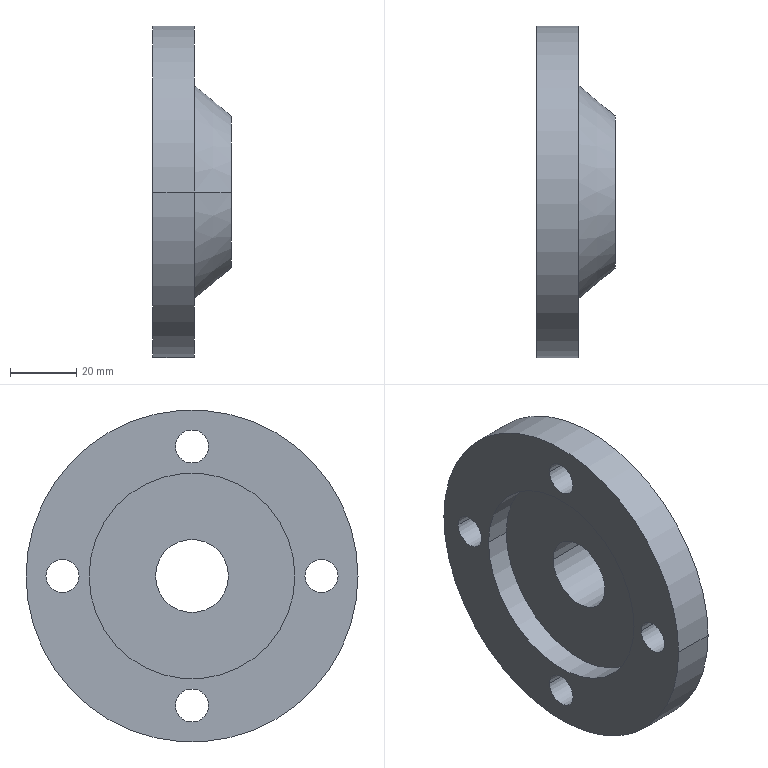Component | SolidWorks | RearEndCap-1 | 1 solid | 20 faces | box 23.63 x 100 x 100 mm | volume 92342 mm3 | cylinder 14 | plane 4 | cone 2 | commonest cylinder face diameters 10 x8 62 x2 100 x2 22 x2
build123d program:
from build123d import *

# Parameters (mm, degrees)
CUT_EXTRUDE1_DEPTH      = 211.672
CUT_EXTRUDE1_DEPTH_BACK = 211.672
SKETCH4_R               = 5
CUT_EXTRUDE2_START      = -5
SKETCH5_R               = 31
CUT_EXTRUDE2_DEPTH      = 10


with BuildPart() as part:
    # Sketch3 → Revolve1 (revolve)
    with BuildSketch(Plane(origin=(15, 0, 0), x_dir=(0, 0, -1), z_dir=(1, 0, 0)), mode=Mode.PRIVATE) as revolve1_sk:
        Polygon((0, 200), (-12.554, 200), (-12.554, 182.147), (-23.63, 172.896), (-23.63, 161), (0, 161), align=None)
    revolve(revolve1_sk.sketch.rotate(Axis((15, 150, 44.24), (0, 0, -1)), 90), axis=Axis((15, 150, 44.24), (0, 0, -1)))

    # Sketch4 → Cut-Extrude1 (cut, two sides: drawn at the far end of the back side and taken through both)
    with BuildSketch(Plane.XY.offset(12.554).offset(-CUT_EXTRUDE1_DEPTH_BACK)):
        with Locations((15, 189)):
            Circle(SKETCH4_R)
        with Locations((54, 150)):
            Circle(SKETCH4_R)
        with Locations((15, 111)):
            Circle(SKETCH4_R)
        with Locations((-24, 150)):
            Circle(SKETCH4_R)
    extrude(amount=CUT_EXTRUDE1_DEPTH + CUT_EXTRUDE1_DEPTH_BACK, mode=Mode.SUBTRACT)

    # Sketch5 → Cut-Extrude2 (cut)
    with BuildSketch(Plane.XY.offset(12.554).offset(CUT_EXTRUDE2_START)):
        with Locations((15, 150)):
            Circle(SKETCH5_R)
    extrude(amount=-CUT_EXTRUDE2_DEPTH, mode=Mode.SUBTRACT)


solid = part.part

# Placed as in the assembly
solid = solid.moved(Location((110, 0, 0), (0, 90, 0)))
STEP:
#1=COLOUR_RGB('',0.7922,0.8196,0.9333);
#2=FILL_AREA_STYLE_COLOUR('',#1);
#3=FILL_AREA_STYLE('',(#2));
#4=SURFACE_STYLE_FILL_AREA(#3);
#5=SURFACE_SIDE_STYLE('',(#4));
#6=SURFACE_STYLE_USAGE(.BOTH.,#5);
#7=PRESENTATION_STYLE_ASSIGNMENT((#6));
#8=CARTESIAN_POINT('',(4.331,7.126,-0.5906));
#9=VERTEX_POINT('',#8);
#10=CARTESIAN_POINT('',(4.331,4.685,-0.5906));
#11=VERTEX_POINT('',#10);
#12=CARTESIAN_POINT('',(4.331,5.906,-0.5906));
#13=DIRECTION('',(1.,0.,0.));
#14=DIRECTION('',(0.,-1.,-0.));
#15=AXIS2_PLACEMENT_3D('',#12,#13,#14);
#16=CIRCLE('',#15,1.22);
#17=EDGE_CURVE('',#9,#11,#16,.T.);
#18=ORIENTED_EDGE('',*,*,#17,.F.);
#19=CARTESIAN_POINT('',(4.628,7.126,-0.5906));
#20=VERTEX_POINT('',#19);
#21=CARTESIAN_POINT('',(4.234,7.126,-0.5906));
#22=DIRECTION('',(1.,0.,0.));
#23=VECTOR('',#22,39.37);
#24=LINE('',#21,#23);
#25=EDGE_CURVE('',#9,#20,#24,.T.);
#26=ORIENTED_EDGE('',*,*,#25,.T.);
#27=CARTESIAN_POINT('',(4.628,4.685,-0.5906));
#28=VERTEX_POINT('',#27);
#29=CARTESIAN_POINT('',(4.628,5.906,-0.5906));
#30=DIRECTION('',(1.,0.,0.));
#31=DIRECTION('',(0.,-1.,-0.));
#32=AXIS2_PLACEMENT_3D('',#29,#30,#31);
#33=CIRCLE('',#32,1.22);
#34=EDGE_CURVE('',#20,#28,#33,.T.);
#35=ORIENTED_EDGE('',*,*,#34,.T.);
#36=CARTESIAN_POINT('',(4.234,4.685,-0.5906));
#37=DIRECTION('',(1.,0.,0.));
#38=VECTOR('',#37,39.37);
#39=LINE('',#36,#38);
#40=EDGE_CURVE('',#11,#28,#39,.T.);
#41=ORIENTED_EDGE('',*,*,#40,.F.);
#42=EDGE_LOOP('',(#18,#26,#35,#41));
#43=FACE_OUTER_BOUND('',#42,.T.);
#44=CARTESIAN_POINT('',(4.234,5.906,-0.5906));
#45=DIRECTION('',(1.,0.,0.));
#46=DIRECTION('',(0.,-1.,-0.));
#47=AXIS2_PLACEMENT_3D('',#44,#45,#46);
#48=CYLINDRICAL_SURFACE('',#47,1.22);
#49=ADVANCED_FACE('',(#43),#48,.F.);
#50=CARTESIAN_POINT('',(4.331,6.102,-2.126));
#51=VERTEX_POINT('',#50);
#52=CARTESIAN_POINT('',(4.331,5.709,-2.126));
#53=VERTEX_POINT('',#52);
#54=CARTESIAN_POINT('',(4.331,5.906,-2.126));
#55=DIRECTION('',(1.,0.,0.));
#56=DIRECTION('',(0.,-1.,-0.));
#57=AXIS2_PLACEMENT_3D('',#54,#55,#56);
#58=CIRCLE('',#57,0.1969);
#59=EDGE_CURVE('',#51,#53,#58,.T.);
#60=ORIENTED_EDGE('',*,*,#59,.F.);
#61=CARTESIAN_POINT('',(4.825,6.102,-2.126));
#62=VERTEX_POINT('',#61);
#63=CARTESIAN_POINT('',(4.331,6.102,-2.126));
#64=DIRECTION('',(1.,0.,0.));
#65=VECTOR('',#64,39.37);
#66=LINE('',#63,#65);
#67=EDGE_CURVE('',#51,#62,#66,.T.);
#68=ORIENTED_EDGE('',*,*,#67,.T.);
#69=CARTESIAN_POINT('',(4.825,5.709,-2.126));
#70=VERTEX_POINT('',#69);
#71=CARTESIAN_POINT('',(4.825,5.906,-2.126));
#72=DIRECTION('',(-1.,-0.,-0.));
#73=DIRECTION('',(0.,1.,0.));
#74=AXIS2_PLACEMENT_3D('',#71,#72,#73);
#75=CIRCLE('',#74,0.1969);
#76=EDGE_CURVE('',#70,#62,#75,.T.);
#77=ORIENTED_EDGE('',*,*,#76,.F.);
#78=CARTESIAN_POINT('',(4.331,5.709,-2.126));
#79=DIRECTION('',(1.,0.,0.));
#80=VECTOR('',#79,39.37);
#81=LINE('',#78,#80);
#82=EDGE_CURVE('',#53,#70,#81,.T.);
#83=ORIENTED_EDGE('',*,*,#82,.F.);
#84=EDGE_LOOP('',(#60,#68,#77,#83));
#85=FACE_OUTER_BOUND('',#84,.T.);
#86=CARTESIAN_POINT('',(4.331,5.906,-2.126));
#87=DIRECTION('',(1.,0.,0.));
#88=DIRECTION('',(0.,-1.,-0.));
#89=AXIS2_PLACEMENT_3D('',#86,#87,#88);
#90=CYLINDRICAL_SURFACE('',#89,0.1969);
#91=ADVANCED_FACE('',(#85),#90,.F.);
#92=CARTESIAN_POINT('',(4.331,4.567,-0.5906));
#93=VERTEX_POINT('',#92);
#94=CARTESIAN_POINT('',(4.331,4.173,-0.5906));
#95=VERTEX_POINT('',#94);
#96=CARTESIAN_POINT('',(4.331,4.37,-0.5906));
#97=DIRECTION('',(1.,0.,0.));
#98=DIRECTION('',(0.,-1.,-0.));
#99=AXIS2_PLACEMENT_3D('',#96,#97,#98);
#100=CIRCLE('',#99,0.1969);
#101=EDGE_CURVE('',#93,#95,#100,.T.);
#102=ORIENTED_EDGE('',*,*,#101,.F.);
#103=CARTESIAN_POINT('',(4.825,4.567,-0.5906));
#104=VERTEX_POINT('',#103);
#105=CARTESIAN_POINT('',(4.331,4.567,-0.5906));
#106=DIRECTION('',(1.,0.,0.));
#107=VECTOR('',#106,39.37);
#108=LINE('',#105,#107);
#109=EDGE_CURVE('',#93,#104,#108,.T.);
#110=ORIENTED_EDGE('',*,*,#109,.T.);
#111=CARTESIAN_POINT('',(4.825,4.173,-0.5906));
#112=VERTEX_POINT('',#111);
#113=CARTESIAN_POINT('',(4.825,4.37,-0.5906));
#114=DIRECTION('',(-1.,-0.,-0.));
#115=DIRECTION('',(0.,1.,0.));
#116=AXIS2_PLACEMENT_3D('',#113,#114,#115);
#117=CIRCLE('',#116,0.1969);
#118=EDGE_CURVE('',#112,#104,#117,.T.);
#119=ORIENTED_EDGE('',*,*,#118,.F.);
#120=CARTESIAN_POINT('',(4.331,4.173,-0.5906));
#121=DIRECTION('',(1.,0.,0.));
#122=VECTOR('',#121,39.37);
#123=LINE('',#120,#122);
#124=EDGE_CURVE('',#95,#112,#123,.T.);
#125=ORIENTED_EDGE('',*,*,#124,.F.);
#126=EDGE_LOOP('',(#102,#110,#119,#125));
#127=FACE_OUTER_BOUND('',#126,.T.);
#128=CARTESIAN_POINT('',(4.331,4.37,-0.5906));
#129=DIRECTION('',(1.,0.,0.));
#130=DIRECTION('',(0.,-1.,-0.));
#131=AXIS2_PLACEMENT_3D('',#128,#129,#130);
#132=CYLINDRICAL_SURFACE('',#131,0.1969);
#133=ADVANCED_FACE('',(#127),#132,.F.);
#134=CARTESIAN_POINT('',(4.331,6.102,0.9449));
#135=VERTEX_POINT('',#134);
#136=CARTESIAN_POINT('',(4.331,5.709,0.9449));
#137=VERTEX_POINT('',#136);
#138=CARTESIAN_POINT('',(4.331,5.906,0.9449));
#139=DIRECTION('',(1.,0.,0.));
#140=DIRECTION('',(0.,-1.,-0.));
#141=AXIS2_PLACEMENT_3D('',#138,#139,#140);
#142=CIRCLE('',#141,0.1969);
#143=EDGE_CURVE('',#135,#137,#142,.T.);
#144=ORIENTED_EDGE('',*,*,#143,.F.);
#145=CARTESIAN_POINT('',(4.825,6.102,0.9449));
#146=VERTEX_POINT('',#145);
#147=CARTESIAN_POINT('',(4.331,6.102,0.9449));
#148=DIRECTION('',(1.,0.,0.));
#149=VECTOR('',#148,39.37);
#150=LINE('',#147,#149);
#151=EDGE_CURVE('',#135,#146,#150,.T.);
#152=ORIENTED_EDGE('',*,*,#151,.T.);
#153=CARTESIAN_POINT('',(4.825,5.709,0.9449));
#154=VERTEX_POINT('',#153);
#155=CARTESIAN_POINT('',(4.825,5.906,0.9449));
#156=DIRECTION('',(-1.,-0.,-0.));
#157=DIRECTION('',(0.,1.,0.));
#158=AXIS2_PLACEMENT_3D('',#155,#156,#157);
#159=CIRCLE('',#158,0.1969);
#160=EDGE_CURVE('',#154,#146,#159,.T.);
#161=ORIENTED_EDGE('',*,*,#160,.F.);
#162=CARTESIAN_POINT('',(4.331,5.709,0.9449));
#163=DIRECTION('',(1.,0.,0.));
#164=VECTOR('',#163,39.37);
#165=LINE('',#162,#164);
#166=EDGE_CURVE('',#137,#154,#165,.T.);
#167=ORIENTED_EDGE('',*,*,#166,.F.);
#168=EDGE_LOOP('',(#144,#152,#161,#167));
#169=FACE_OUTER_BOUND('',#168,.T.);
#170=CARTESIAN_POINT('',(4.331,5.906,0.9449));
#171=DIRECTION('',(1.,0.,0.));
#172=DIRECTION('',(0.,-1.,-0.));
#173=AXIS2_PLACEMENT_3D('',#170,#171,#172);
#174=CYLINDRICAL_SURFACE('',#173,0.1969);
#175=ADVANCED_FACE('',(#169),#174,.F.);
#176=CARTESIAN_POINT('',(4.331,7.638,-0.5906));
#177=VERTEX_POINT('',#176);
#178=CARTESIAN_POINT('',(4.331,7.244,-0.5906));
#179=VERTEX_POINT('',#178);
#180=CARTESIAN_POINT('',(4.331,7.441,-0.5906));
#181=DIRECTION('',(1.,0.,0.));
#182=DIRECTION('',(0.,-1.,-0.));
#183=AXIS2_PLACEMENT_3D('',#180,#181,#182);
#184=CIRCLE('',#183,0.1969);
#185=EDGE_CURVE('',#177,#179,#184,.T.);
#186=ORIENTED_EDGE('',*,*,#185,.F.);
#187=CARTESIAN_POINT('',(4.825,7.638,-0.5906));
#188=VERTEX_POINT('',#187);
#189=CARTESIAN_POINT('',(4.331,7.638,-0.5906));
#190=DIRECTION('',(1.,0.,0.));
#191=VECTOR('',#190,39.37);
#192=LINE('',#189,#191);
#193=EDGE_CURVE('',#177,#188,#192,.T.);
#194=ORIENTED_EDGE('',*,*,#193,.T.);
#195=CARTESIAN_POINT('',(4.825,7.244,-0.5906));
#196=VERTEX_POINT('',#195);
#197=CARTESIAN_POINT('',(4.825,7.441,-0.5906));
#198=DIRECTION('',(-1.,-0.,-0.));
#199=DIRECTION('',(0.,1.,0.));
#200=AXIS2_PLACEMENT_3D('',#197,#198,#199);
#201=CIRCLE('',#200,0.1969);
#202=EDGE_CURVE('',#196,#188,#201,.T.);
#203=ORIENTED_EDGE('',*,*,#202,.F.);
#204=CARTESIAN_POINT('',(4.331,7.244,-0.5906));
#205=DIRECTION('',(1.,0.,0.));
#206=VECTOR('',#205,39.37);
#207=LINE('',#204,#206);
#208=EDGE_CURVE('',#179,#196,#207,.T.);
#209=ORIENTED_EDGE('',*,*,#208,.F.);
#210=EDGE_LOOP('',(#186,#194,#203,#209));
#211=FACE_OUTER_BOUND('',#210,.T.);
#212=CARTESIAN_POINT('',(4.331,7.441,-0.5906));
#213=DIRECTION('',(1.,0.,0.));
#214=DIRECTION('',(0.,-1.,-0.));
#215=AXIS2_PLACEMENT_3D('',#212,#213,#214);
#216=CYLINDRICAL_SURFACE('',#215,0.1969);
#217=ADVANCED_FACE('',(#211),#216,.F.);
#218=CARTESIAN_POINT('',(4.331,3.937,-0.5906));
#219=VERTEX_POINT('',#218);
#220=CARTESIAN_POINT('',(4.331,7.874,-0.5906));
#221=VERTEX_POINT('',#220);
#222=CARTESIAN_POINT('',(4.331,5.906,-0.5906));
#223=DIRECTION('',(1.,0.,0.));
#224=DIRECTION('',(0.,-1.,-0.));
#225=AXIS2_PLACEMENT_3D('',#222,#223,#224);
#226=CIRCLE('',#225,1.969);
#227=EDGE_CURVE('',#219,#221,#226,.T.);
#228=ORIENTED_EDGE('',*,*,#227,.T.);
#229=CARTESIAN_POINT('',(4.825,7.874,-0.5906));
#230=VERTEX_POINT('',#229);
#231=CARTESIAN_POINT('',(6.072,7.874,-0.5906));
#232=DIRECTION('',(1.,0.,0.));
#233=VECTOR('',#232,39.37);
#234=LINE('',#231,#233);
#235=EDGE_CURVE('',#221,#230,#234,.T.);
#236=ORIENTED_EDGE('',*,*,#235,.T.);
#237=CARTESIAN_POINT('',(4.825,3.937,-0.5906));
#238=VERTEX_POINT('',#237);
#239=CARTESIAN_POINT('',(4.825,5.906,-0.5906));
#240=DIRECTION('',(1.,0.,0.));
#241=DIRECTION('',(0.,-1.,-0.));
#242=AXIS2_PLACEMENT_3D('',#239,#240,#241);
#243=CIRCLE('',#242,1.969);
#244=EDGE_CURVE('',#238,#230,#243,.T.);
#245=ORIENTED_EDGE('',*,*,#244,.F.);
#246=CARTESIAN_POINT('',(6.072,3.937,-0.5906));
#247=DIRECTION('',(1.,0.,0.));
#248=VECTOR('',#247,39.37);
#249=LINE('',#246,#248);
#250=EDGE_CURVE('',#219,#238,#249,.T.);
#251=ORIENTED_EDGE('',*,*,#250,.F.);
#252=EDGE_LOOP('',(#228,#236,#245,#251));
#253=FACE_OUTER_BOUND('',#252,.T.);
#254=CARTESIAN_POINT('',(6.072,5.906,-0.5906));
#255=DIRECTION('',(1.,0.,0.));
#256=DIRECTION('',(0.,-1.,-0.));
#257=AXIS2_PLACEMENT_3D('',#254,#255,#256);
#258=CYLINDRICAL_SURFACE('',#257,1.969);
#259=ADVANCED_FACE('',(#253),#258,.T.);
#260=CARTESIAN_POINT('',(5.261,5.004,-0.5906));
#261=VERTEX_POINT('',#260);
#262=CARTESIAN_POINT('',(5.261,6.807,-0.5906));
#263=VERTEX_POINT('',#262);
#264=CARTESIAN_POINT('',(5.261,5.906,-0.5906));
#265=DIRECTION('',(1.,0.,0.));
#266=DIRECTION('',(0.,-1.,-0.));
#267=AXIS2_PLACEMENT_3D('',#264,#265,#266);
#268=CIRCLE('',#267,0.9014);
#269=EDGE_CURVE('',#261,#263,#268,.T.);
#270=ORIENTED_EDGE('',*,*,#269,.F.);
#271=CARTESIAN_POINT('',(4.825,4.64,-0.5906));
#272=VERTEX_POINT('',#271);
#273=CARTESIAN_POINT('',(4.825,4.64,-0.5906));
#274=DIRECTION('',(-0.7675,-0.641,-0.));
#275=VECTOR('',#274,39.37);
#276=LINE('',#273,#275);
#277=EDGE_CURVE('',#261,#272,#276,.T.);
#278=ORIENTED_EDGE('',*,*,#277,.T.);
#279=CARTESIAN_POINT('',(4.825,7.171,-0.5906));
#280=VERTEX_POINT('',#279);
#281=CARTESIAN_POINT('',(4.825,5.906,-0.5906));
#282=DIRECTION('',(1.,0.,0.));
#283=DIRECTION('',(0.,-1.,-0.));
#284=AXIS2_PLACEMENT_3D('',#281,#282,#283);
#285=CIRCLE('',#284,1.266);
#286=EDGE_CURVE('',#272,#280,#285,.T.);
#287=ORIENTED_EDGE('',*,*,#286,.T.);
#288=CARTESIAN_POINT('',(4.825,7.171,-0.5906));
#289=DIRECTION('',(-0.7675,0.641,0.));
#290=VECTOR('',#289,39.37);
#291=LINE('',#288,#290);
#292=EDGE_CURVE('',#263,#280,#291,.T.);
#293=ORIENTED_EDGE('',*,*,#292,.F.);
#294=EDGE_LOOP('',(#270,#278,#287,#293));
#295=FACE_OUTER_BOUND('',#294,.T.);
#296=CARTESIAN_POINT('',(4.825,5.906,-0.5906));
#297=DIRECTION('',(-1.,-0.,-0.));
#298=DIRECTION('',(0.,1.,0.));
#299=AXIS2_PLACEMENT_3D('',#296,#297,#298);
#300=CONICAL_SURFACE('',#299,1.266,0.6959);
#301=ADVANCED_FACE('',(#295),#300,.T.);
#302=CARTESIAN_POINT('',(4.628,5.472,-0.5906));
#303=VERTEX_POINT('',#302);
#304=CARTESIAN_POINT('',(4.628,6.339,-0.5906));
#305=VERTEX_POINT('',#304);
#306=CARTESIAN_POINT('',(4.628,5.906,-0.5906));
#307=DIRECTION('',(-1.,-0.,-0.));
#308=DIRECTION('',(0.,-1.,-0.));
#309=AXIS2_PLACEMENT_3D('',#306,#307,#308);
#310=CIRCLE('',#309,0.4331);
#311=EDGE_CURVE('',#303,#305,#310,.T.);
#312=ORIENTED_EDGE('',*,*,#311,.T.);
#313=CARTESIAN_POINT('',(5.261,6.339,-0.5906));
#314=VERTEX_POINT('',#313);
#315=CARTESIAN_POINT('',(6.072,6.339,-0.5906));
#316=DIRECTION('',(1.,0.,0.));
#317=VECTOR('',#316,39.37);
#318=LINE('',#315,#317);
#319=EDGE_CURVE('',#305,#314,#318,.T.);
#320=ORIENTED_EDGE('',*,*,#319,.T.);
#321=CARTESIAN_POINT('',(5.261,5.472,-0.5906));
#322=VERTEX_POINT('',#321);
#323=CARTESIAN_POINT('',(5.261,5.906,-0.5906));
#324=DIRECTION('',(1.,0.,0.));
#325=DIRECTION('',(0.,-1.,-0.));
#326=AXIS2_PLACEMENT_3D('',#323,#324,#325);
#327=CIRCLE('',#326,0.4331);
#328=EDGE_CURVE('',#314,#322,#327,.T.);
#329=ORIENTED_EDGE('',*,*,#328,.T.);
#330=CARTESIAN_POINT('',(6.072,5.472,-0.5906));
#331=DIRECTION('',(1.,0.,0.));
#332=VECTOR('',#331,39.37);
#333=LINE('',#330,#332);
#334=EDGE_CURVE('',#303,#322,#333,.T.);
#335=ORIENTED_EDGE('',*,*,#334,.F.);
#336=EDGE_LOOP('',(#312,#320,#329,#335));
#337=FACE_OUTER_BOUND('',#336,.T.);
#338=CARTESIAN_POINT('',(6.072,5.906,-0.5906));
#339=DIRECTION('',(1.,0.,0.));
#340=DIRECTION('',(0.,-1.,-0.));
#341=AXIS2_PLACEMENT_3D('',#338,#339,#340);
#342=CYLINDRICAL_SURFACE('',#341,0.4331);
#343=ADVANCED_FACE('',(#337),#342,.F.);
#344=CARTESIAN_POINT('',(4.331,5.906,-0.5906));
#345=DIRECTION('',(1.,0.,0.));
#346=DIRECTION('',(0.,-1.,-0.));
#347=AXIS2_PLACEMENT_3D('',#344,#345,#346);
#348=CIRCLE('',#347,1.22);
#349=EDGE_CURVE('',#11,#9,#348,.T.);
#350=ORIENTED_EDGE('',*,*,#349,.T.);
#351=ORIENTED_EDGE('',*,*,#17,.T.);
#352=EDGE_LOOP('',(#350,#351));
#353=FACE_BOUND('',#352,.T.);
#354=CARTESIAN_POINT('',(4.331,5.906,-2.126));
#355=DIRECTION('',(1.,0.,0.));
#356=DIRECTION('',(0.,-1.,-0.));
#357=AXIS2_PLACEMENT_3D('',#354,#355,#356);
#358=CIRCLE('',#357,0.1969);
#359=EDGE_CURVE('',#53,#51,#358,.T.);
#360=ORIENTED_EDGE('',*,*,#359,.T.);
#361=ORIENTED_EDGE('',*,*,#59,.T.);
#362=EDGE_LOOP('',(#360,#361));
#363=FACE_BOUND('',#362,.T.);
#364=CARTESIAN_POINT('',(4.331,4.37,-0.5906));
#365=DIRECTION('',(1.,0.,0.));
#366=DIRECTION('',(0.,-1.,-0.));
#367=AXIS2_PLACEMENT_3D('',#364,#365,#366);
#368=CIRCLE('',#367,0.1969);
#369=EDGE_CURVE('',#95,#93,#368,.T.);
#370=ORIENTED_EDGE('',*,*,#369,.T.);
#371=ORIENTED_EDGE('',*,*,#101,.T.);
#372=EDGE_LOOP('',(#370,#371));
#373=FACE_BOUND('',#372,.T.);
#374=CARTESIAN_POINT('',(4.331,5.906,0.9449));
#375=DIRECTION('',(1.,0.,0.));
#376=DIRECTION('',(0.,-1.,-0.));
#377=AXIS2_PLACEMENT_3D('',#374,#375,#376);
#378=CIRCLE('',#377,0.1969);
#379=EDGE_CURVE('',#137,#135,#378,.T.);
#380=ORIENTED_EDGE('',*,*,#379,.T.);
#381=ORIENTED_EDGE('',*,*,#143,.T.);
#382=EDGE_LOOP('',(#380,#381));
#383=FACE_BOUND('',#382,.T.);
#384=CARTESIAN_POINT('',(4.331,7.441,-0.5906));
#385=DIRECTION('',(1.,0.,0.));
#386=DIRECTION('',(0.,-1.,-0.));
#387=AXIS2_PLACEMENT_3D('',#384,#385,#386);
#388=CIRCLE('',#387,0.1969);
#389=EDGE_CURVE('',#179,#177,#388,.T.);
#390=ORIENTED_EDGE('',*,*,#389,.T.);
#391=ORIENTED_EDGE('',*,*,#185,.T.);
#392=EDGE_LOOP('',(#390,#391));
#393=FACE_BOUND('',#392,.T.);
#394=ORIENTED_EDGE('',*,*,#227,.F.);
#395=CARTESIAN_POINT('',(4.331,5.906,-0.5906));
#396=DIRECTION('',(1.,0.,0.));
#397=DIRECTION('',(0.,-1.,-0.));
#398=AXIS2_PLACEMENT_3D('',#395,#396,#397);
#399=CIRCLE('',#398,1.969);
#400=EDGE_CURVE('',#221,#219,#399,.T.);
#401=ORIENTED_EDGE('',*,*,#400,.F.);
#402=EDGE_LOOP('',(#394,#401));
#403=FACE_OUTER_BOUND('',#402,.T.);
#404=CARTESIAN_POINT('',(4.331,5.906,-2.559));
#405=DIRECTION('',(1.,0.,0.));
#406=DIRECTION('',(0.,-1.,-0.));
#407=AXIS2_PLACEMENT_3D('',#404,#405,#406);
#408=PLANE('',#407);
#409=ADVANCED_FACE('',(#353,#363,#373,#383,#393,#403),#408,.F.);
#410=ORIENTED_EDGE('',*,*,#319,.F.);
#411=CARTESIAN_POINT('',(4.628,5.906,-0.5906));
#412=DIRECTION('',(-1.,-0.,-0.));
#413=DIRECTION('',(0.,-1.,-0.));
#414=AXIS2_PLACEMENT_3D('',#411,#412,#413);
#415=CIRCLE('',#414,0.4331);
#416=EDGE_CURVE('',#305,#303,#415,.T.);
#417=ORIENTED_EDGE('',*,*,#416,.T.);
#418=ORIENTED_EDGE('',*,*,#334,.T.);
#419=CARTESIAN_POINT('',(5.261,5.906,-0.5906));
#420=DIRECTION('',(1.,0.,0.));
#421=DIRECTION('',(0.,-1.,-0.));
#422=AXIS2_PLACEMENT_3D('',#419,#420,#421);
#423=CIRCLE('',#422,0.4331);
#424=EDGE_CURVE('',#322,#314,#423,.T.);
#425=ORIENTED_EDGE('',*,*,#424,.T.);
#426=EDGE_LOOP('',(#410,#417,#418,#425));
#427=FACE_OUTER_BOUND('',#426,.T.);
#428=CARTESIAN_POINT('',(6.072,5.906,-0.5906));
#429=DIRECTION('',(1.,0.,0.));
#430=DIRECTION('',(0.,-1.,-0.));
#431=AXIS2_PLACEMENT_3D('',#428,#429,#430);
#432=CYLINDRICAL_SURFACE('',#431,0.4331);
#433=ADVANCED_FACE('',(#427),#432,.F.);
#434=ORIENTED_EDGE('',*,*,#424,.F.);
#435=ORIENTED_EDGE('',*,*,#328,.F.);
#436=EDGE_LOOP('',(#434,#435));
#437=FACE_BOUND('',#436,.T.);
#438=CARTESIAN_POINT('',(5.261,5.906,-0.5906));
#439=DIRECTION('',(1.,0.,0.));
#440=DIRECTION('',(0.,-1.,-0.));
#441=AXIS2_PLACEMENT_3D('',#438,#439,#440);
#442=CIRCLE('',#441,0.9014);
#443=EDGE_CURVE('',#263,#261,#442,.T.);
#444=ORIENTED_EDGE('',*,*,#443,.T.);
#445=ORIENTED_EDGE('',*,*,#269,.T.);
#446=EDGE_LOOP('',(#444,#445));
#447=FACE_OUTER_BOUND('',#446,.T.);
#448=CARTESIAN_POINT('',(5.261,5.906,-1.492));
#449=DIRECTION('',(-1.,-0.,-0.));
#450=DIRECTION('',(-0.,1.,0.));
#451=AXIS2_PLACEMENT_3D('',#448,#449,#450);
#452=PLANE('',#451);
#453=ADVANCED_FACE('',(#437,#447),#452,.F.);
#454=ORIENTED_EDGE('',*,*,#277,.F.);
#455=ORIENTED_EDGE('',*,*,#443,.F.);
#456=ORIENTED_EDGE('',*,*,#292,.T.);
#457=CARTESIAN_POINT('',(4.825,5.906,-0.5906));
#458=DIRECTION('',(1.,0.,0.));
#459=DIRECTION('',(0.,-1.,-0.));
#460=AXIS2_PLACEMENT_3D('',#457,#458,#459);
#461=CIRCLE('',#460,1.266);
#462=EDGE_CURVE('',#280,#272,#461,.T.);
#463=ORIENTED_EDGE('',*,*,#462,.T.);
#464=EDGE_LOOP('',(#454,#455,#456,#463));
#465=FACE_OUTER_BOUND('',#464,.T.);
#466=CARTESIAN_POINT('',(4.825,5.906,-0.5906));
#467=DIRECTION('',(-1.,-0.,-0.));
#468=DIRECTION('',(0.,1.,0.));
#469=AXIS2_PLACEMENT_3D('',#466,#467,#468);
#470=CONICAL_SURFACE('',#469,1.266,0.6959);
#471=ADVANCED_FACE('',(#465),#470,.T.);
#472=ORIENTED_EDGE('',*,*,#76,.T.);
#473=CARTESIAN_POINT('',(4.825,5.906,-2.126));
#474=DIRECTION('',(-1.,-0.,-0.));
#475=DIRECTION('',(0.,1.,0.));
#476=AXIS2_PLACEMENT_3D('',#473,#474,#475);
#477=CIRCLE('',#476,0.1969);
#478=EDGE_CURVE('',#62,#70,#477,.T.);
#479=ORIENTED_EDGE('',*,*,#478,.T.);
#480=EDGE_LOOP('',(#472,#479));
#481=FACE_BOUND('',#480,.T.);
#482=ORIENTED_EDGE('',*,*,#118,.T.);
#483=CARTESIAN_POINT('',(4.825,4.37,-0.5906));
#484=DIRECTION('',(-1.,-0.,-0.));
#485=DIRECTION('',(0.,1.,0.));
#486=AXIS2_PLACEMENT_3D('',#483,#484,#485);
#487=CIRCLE('',#486,0.1969);
#488=EDGE_CURVE('',#104,#112,#487,.T.);
#489=ORIENTED_EDGE('',*,*,#488,.T.);
#490=EDGE_LOOP('',(#482,#489));
#491=FACE_BOUND('',#490,.T.);
#492=ORIENTED_EDGE('',*,*,#160,.T.);
#493=CARTESIAN_POINT('',(4.825,5.906,0.9449));
#494=DIRECTION('',(-1.,-0.,-0.));
#495=DIRECTION('',(0.,1.,0.));
#496=AXIS2_PLACEMENT_3D('',#493,#494,#495);
#497=CIRCLE('',#496,0.1969);
#498=EDGE_CURVE('',#146,#154,#497,.T.);
#499=ORIENTED_EDGE('',*,*,#498,.T.);
#500=EDGE_LOOP('',(#492,#499));
#501=FACE_BOUND('',#500,.T.);
#502=ORIENTED_EDGE('',*,*,#202,.T.);
#503=CARTESIAN_POINT('',(4.825,7.441,-0.5906));
#504=DIRECTION('',(-1.,-0.,-0.));
#505=DIRECTION('',(0.,1.,0.));
#506=AXIS2_PLACEMENT_3D('',#503,#504,#505);
#507=CIRCLE('',#506,0.1969);
#508=EDGE_CURVE('',#188,#196,#507,.T.);
#509=ORIENTED_EDGE('',*,*,#508,.T.);
#510=EDGE_LOOP('',(#502,#509));
#511=FACE_BOUND('',#510,.T.);
#512=ORIENTED_EDGE('',*,*,#462,.F.);
#513=ORIENTED_EDGE('',*,*,#286,.F.);
#514=EDGE_LOOP('',(#512,#513));
#515=FACE_BOUND('',#514,.T.);
#516=ORIENTED_EDGE('',*,*,#244,.T.);
#517=CARTESIAN_POINT('',(4.825,5.906,-0.5906));
#518=DIRECTION('',(1.,0.,0.));
#519=DIRECTION('',(0.,-1.,-0.));
#520=AXIS2_PLACEMENT_3D('',#517,#518,#519);
#521=CIRCLE('',#520,1.969);
#522=EDGE_CURVE('',#230,#238,#521,.T.);
#523=ORIENTED_EDGE('',*,*,#522,.T.);
#524=EDGE_LOOP('',(#516,#523));
#525=FACE_OUTER_BOUND('',#524,.T.);
#526=CARTESIAN_POINT('',(4.825,5.906,-2.559));
#527=DIRECTION('',(-1.,-0.,-0.));
#528=DIRECTION('',(-0.,1.,0.));
#529=AXIS2_PLACEMENT_3D('',#526,#527,#528);
#530=PLANE('',#529);
#531=ADVANCED_FACE('',(#481,#491,#501,#511,#515,#525),#530,.F.);
#532=ORIENTED_EDGE('',*,*,#235,.F.);
#533=ORIENTED_EDGE('',*,*,#400,.T.);
#534=ORIENTED_EDGE('',*,*,#250,.T.);
#535=ORIENTED_EDGE('',*,*,#522,.F.);
#536=EDGE_LOOP('',(#532,#533,#534,#535));
#537=FACE_OUTER_BOUND('',#536,.T.);
#538=CARTESIAN_POINT('',(6.072,5.906,-0.5906));
#539=DIRECTION('',(1.,0.,0.));
#540=DIRECTION('',(0.,-1.,-0.));
#541=AXIS2_PLACEMENT_3D('',#538,#539,#540);
#542=CYLINDRICAL_SURFACE('',#541,1.969);
#543=ADVANCED_FACE('',(#537),#542,.T.);
#544=ORIENTED_EDGE('',*,*,#193,.F.);
#545=ORIENTED_EDGE('',*,*,#389,.F.);
#546=ORIENTED_EDGE('',*,*,#208,.T.);
#547=ORIENTED_EDGE('',*,*,#508,.F.);
#548=EDGE_LOOP('',(#544,#545,#546,#547));
#549=FACE_OUTER_BOUND('',#548,.T.);
#550=CARTESIAN_POINT('',(4.331,7.441,-0.5906));
#551=DIRECTION('',(1.,0.,0.));
#552=DIRECTION('',(0.,-1.,-0.));
#553=AXIS2_PLACEMENT_3D('',#550,#551,#552);
#554=CYLINDRICAL_SURFACE('',#553,0.1969);
#555=ADVANCED_FACE('',(#549),#554,.F.);
#556=ORIENTED_EDGE('',*,*,#151,.F.);
#557=ORIENTED_EDGE('',*,*,#379,.F.);
#558=ORIENTED_EDGE('',*,*,#166,.T.);
#559=ORIENTED_EDGE('',*,*,#498,.F.);
#560=EDGE_LOOP('',(#556,#557,#558,#559));
#561=FACE_OUTER_BOUND('',#560,.T.);
#562=CARTESIAN_POINT('',(4.331,5.906,0.9449));
#563=DIRECTION('',(1.,0.,0.));
#564=DIRECTION('',(0.,-1.,-0.));
#565=AXIS2_PLACEMENT_3D('',#562,#563,#564);
#566=CYLINDRICAL_SURFACE('',#565,0.1969);
#567=ADVANCED_FACE('',(#561),#566,.F.);
#568=ORIENTED_EDGE('',*,*,#109,.F.);
#569=ORIENTED_EDGE('',*,*,#369,.F.);
#570=ORIENTED_EDGE('',*,*,#124,.T.);
#571=ORIENTED_EDGE('',*,*,#488,.F.);
#572=EDGE_LOOP('',(#568,#569,#570,#571));
#573=FACE_OUTER_BOUND('',#572,.T.);
#574=CARTESIAN_POINT('',(4.331,4.37,-0.5906));
#575=DIRECTION('',(1.,0.,0.));
#576=DIRECTION('',(0.,-1.,-0.));
#577=AXIS2_PLACEMENT_3D('',#574,#575,#576);
#578=CYLINDRICAL_SURFACE('',#577,0.1969);
#579=ADVANCED_FACE('',(#573),#578,.F.);
#580=ORIENTED_EDGE('',*,*,#67,.F.);
#581=ORIENTED_EDGE('',*,*,#359,.F.);
#582=ORIENTED_EDGE('',*,*,#82,.T.);
#583=ORIENTED_EDGE('',*,*,#478,.F.);
#584=EDGE_LOOP('',(#580,#581,#582,#583));
#585=FACE_OUTER_BOUND('',#584,.T.);
#586=CARTESIAN_POINT('',(4.331,5.906,-2.126));
#587=DIRECTION('',(1.,0.,0.));
#588=DIRECTION('',(0.,-1.,-0.));
#589=AXIS2_PLACEMENT_3D('',#586,#587,#588);
#590=CYLINDRICAL_SURFACE('',#589,0.1969);
#591=ADVANCED_FACE('',(#585),#590,.F.);
#592=ORIENTED_EDGE('',*,*,#25,.F.);
#593=ORIENTED_EDGE('',*,*,#349,.F.);
#594=ORIENTED_EDGE('',*,*,#40,.T.);
#595=CARTESIAN_POINT('',(4.628,5.906,-0.5906));
#596=DIRECTION('',(1.,0.,0.));
#597=DIRECTION('',(0.,-1.,-0.));
#598=AXIS2_PLACEMENT_3D('',#595,#596,#597);
#599=CIRCLE('',#598,1.22);
#600=EDGE_CURVE('',#28,#20,#599,.T.);
#601=ORIENTED_EDGE('',*,*,#600,.T.);
#602=EDGE_LOOP('',(#592,#593,#594,#601));
#603=FACE_OUTER_BOUND('',#602,.T.);
#604=CARTESIAN_POINT('',(4.234,5.906,-0.5906));
#605=DIRECTION('',(1.,0.,0.));
#606=DIRECTION('',(0.,-1.,-0.));
#607=AXIS2_PLACEMENT_3D('',#604,#605,#606);
#608=CYLINDRICAL_SURFACE('',#607,1.22);
#609=ADVANCED_FACE('',(#603),#608,.F.);
#610=ORIENTED_EDGE('',*,*,#600,.F.);
#611=ORIENTED_EDGE('',*,*,#34,.F.);
#612=EDGE_LOOP('',(#610,#611));
#613=FACE_OUTER_BOUND('',#612,.T.);
#614=ORIENTED_EDGE('',*,*,#311,.F.);
#615=ORIENTED_EDGE('',*,*,#416,.F.);
#616=EDGE_LOOP('',(#614,#615));
#617=FACE_BOUND('',#616,.T.);
#618=CARTESIAN_POINT('',(4.628,5.906,-0.5906));
#619=DIRECTION('',(1.,0.,0.));
#620=DIRECTION('',(0.,-1.,-0.));
#621=AXIS2_PLACEMENT_3D('',#618,#619,#620);
#622=PLANE('',#621);
#623=ADVANCED_FACE('',(#613,#617),#622,.F.);
#624=CLOSED_SHELL('',(#49,#91,#133,#175,#217,#259,#301,#343,#409,#433,#453,#471,#531,#543,#555,#567,#579,#591,#609,#623));
#625=MANIFOLD_SOLID_BREP('',#624);
#626=STYLED_ITEM('',(#7),#625);
#627=PRESENTATION_LAYER_ASSIGNMENT('','',(#626));
#628=(LENGTH_UNIT()NAMED_UNIT(*)SI_UNIT($,.METRE.));
#629=LENGTH_MEASURE_WITH_UNIT(LENGTH_MEASURE(0.0254),#628);
#630=DIMENSIONAL_EXPONENTS(1.,0.,0.,0.,0.,0.,0.);
#631=(CONVERSION_BASED_UNIT('',#629)LENGTH_UNIT()NAMED_UNIT(#630));
#632=UNCERTAINTY_MEASURE_WITH_UNIT(LENGTH_MEASURE(0.00001),#631,'','');
#633=(NAMED_UNIT(*)PLANE_ANGLE_UNIT()SI_UNIT($,.RADIAN.));
#634=(NAMED_UNIT(*)SI_UNIT($,.STERADIAN.)SOLID_ANGLE_UNIT());
#635=(GEOMETRIC_REPRESENTATION_CONTEXT(3)GLOBAL_UNCERTAINTY_ASSIGNED_CONTEXT((#632))GLOBAL_UNIT_ASSIGNED_CONTEXT((#631,#633,#634))REPRESENTATION_CONTEXT('',''));
#636=MECHANICAL_DESIGN_GEOMETRIC_PRESENTATION_REPRESENTATION('',(#626),#635);
#637=CARTESIAN_POINT('',(0.,0.,0.));
#638=DIRECTION('',(0.,0.,1.));
#639=DIRECTION('',(1.,0.,0.));
#640=AXIS2_PLACEMENT_3D('',#637,#638,#639);
#641=(LENGTH_UNIT()NAMED_UNIT(*)SI_UNIT($,.METRE.));
#642=LENGTH_MEASURE_WITH_UNIT(LENGTH_MEASURE(0.0254),#641);
#643=DIMENSIONAL_EXPONENTS(1.,0.,0.,0.,0.,0.,0.);
#644=(CONVERSION_BASED_UNIT('',#642)LENGTH_UNIT()NAMED_UNIT(#643));
#645=UNCERTAINTY_MEASURE_WITH_UNIT(LENGTH_MEASURE(0.00001),#644,'','');
#646=(NAMED_UNIT(*)PLANE_ANGLE_UNIT()SI_UNIT($,.RADIAN.));
#647=(NAMED_UNIT(*)SI_UNIT($,.STERADIAN.)SOLID_ANGLE_UNIT());
#648=(GEOMETRIC_REPRESENTATION_CONTEXT(3)GLOBAL_UNCERTAINTY_ASSIGNED_CONTEXT((#645))GLOBAL_UNIT_ASSIGNED_CONTEXT((#644,#646,#647))REPRESENTATION_CONTEXT('',''));
#649=ADVANCED_BREP_SHAPE_REPRESENTATION('',(#625,#640),#648);